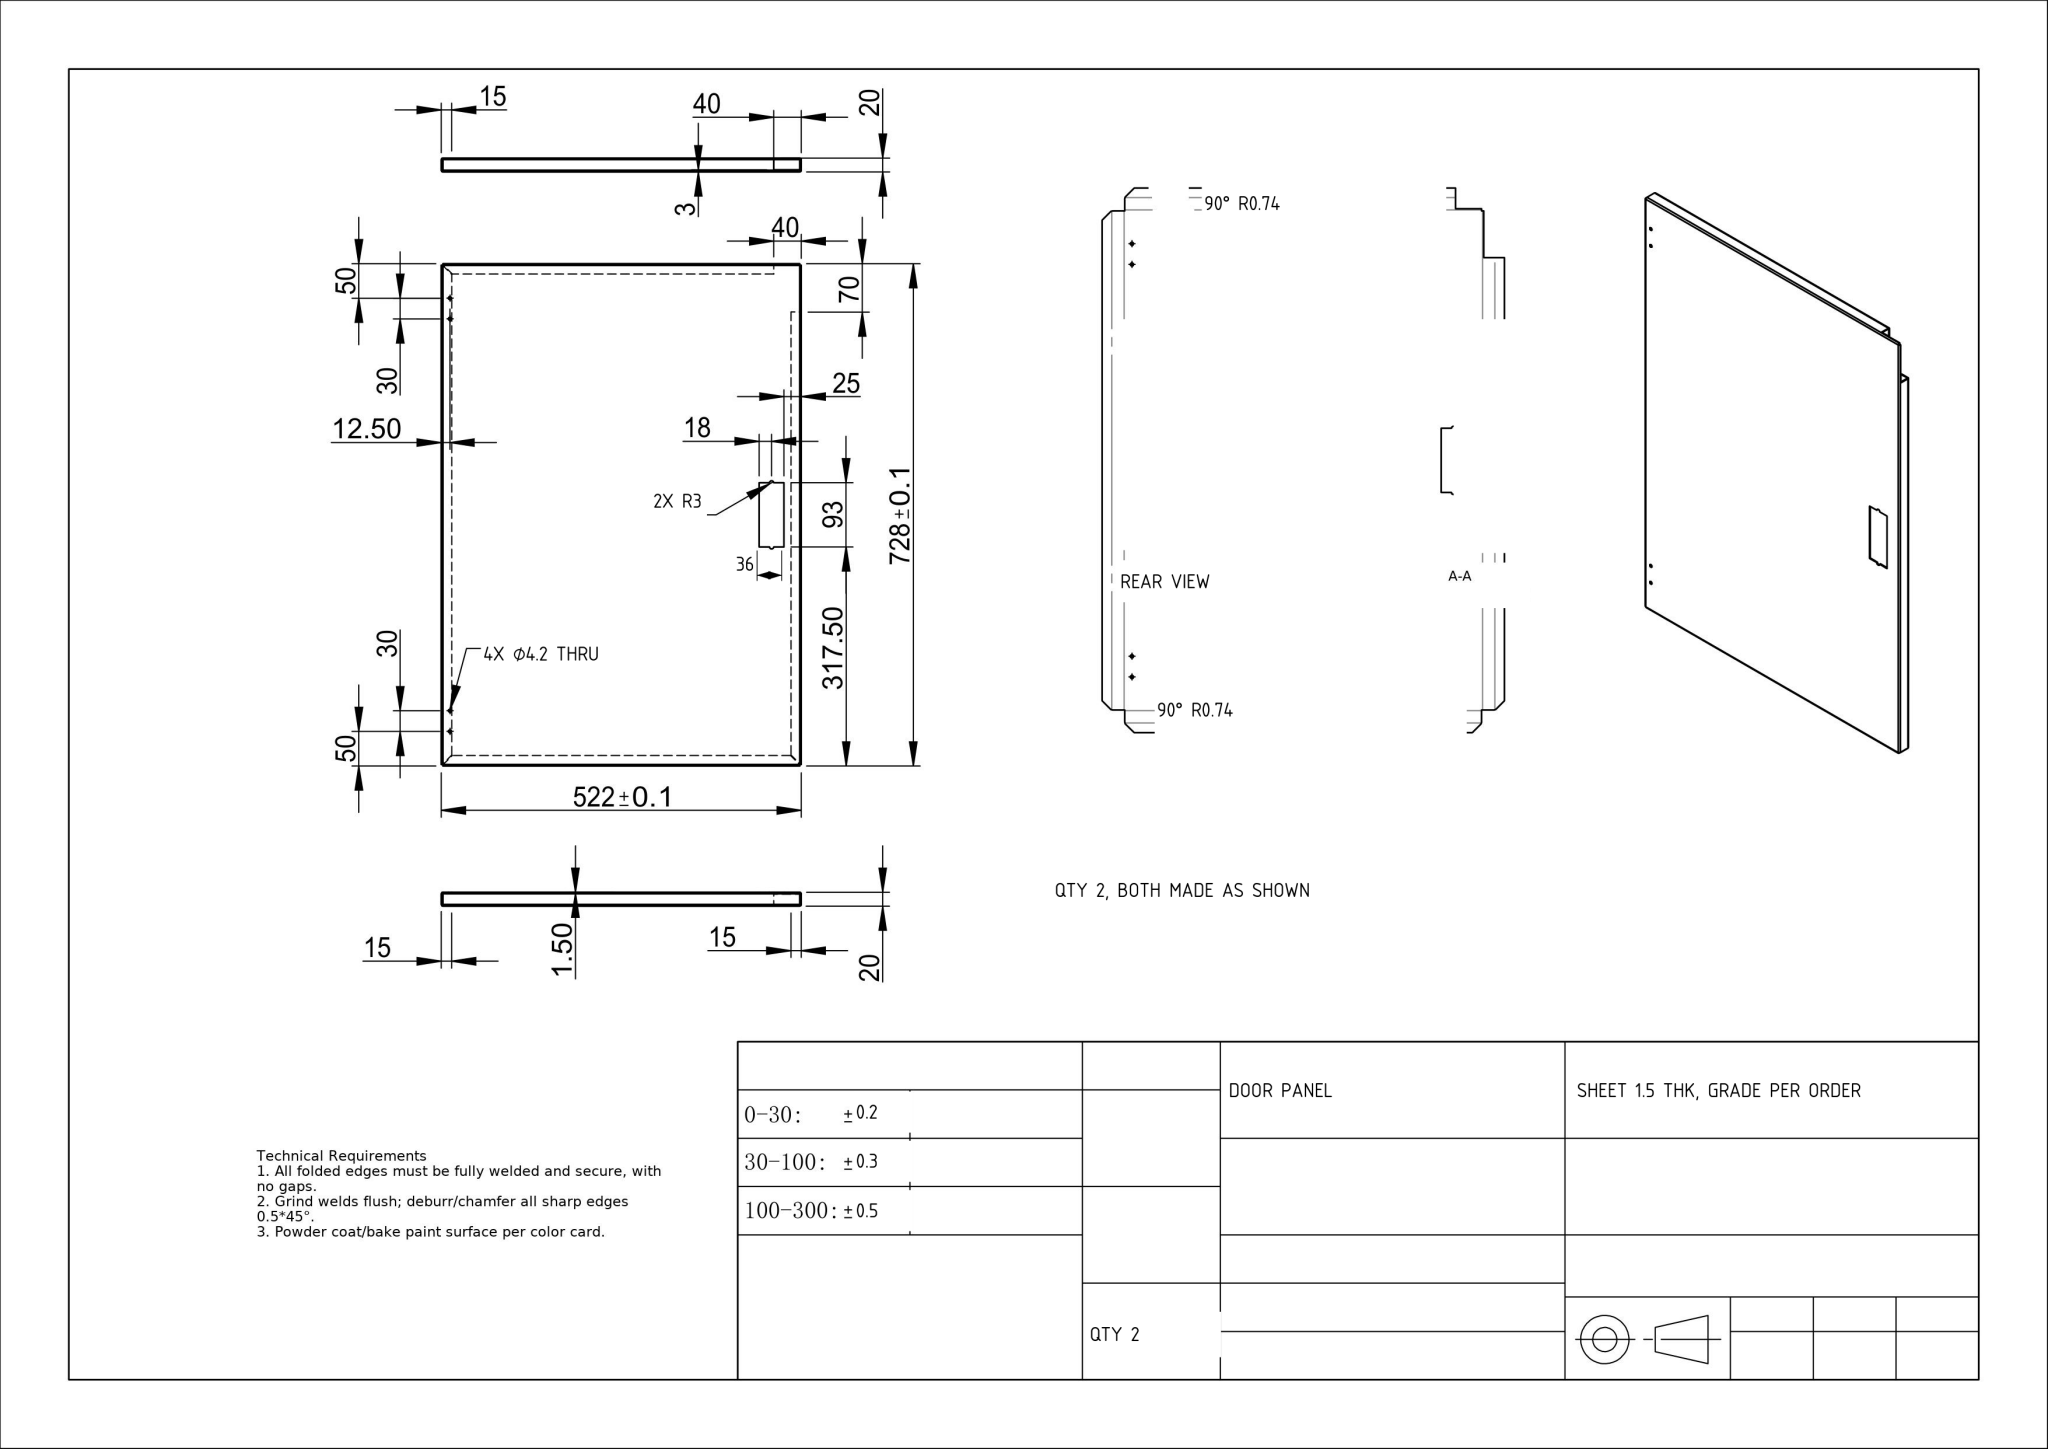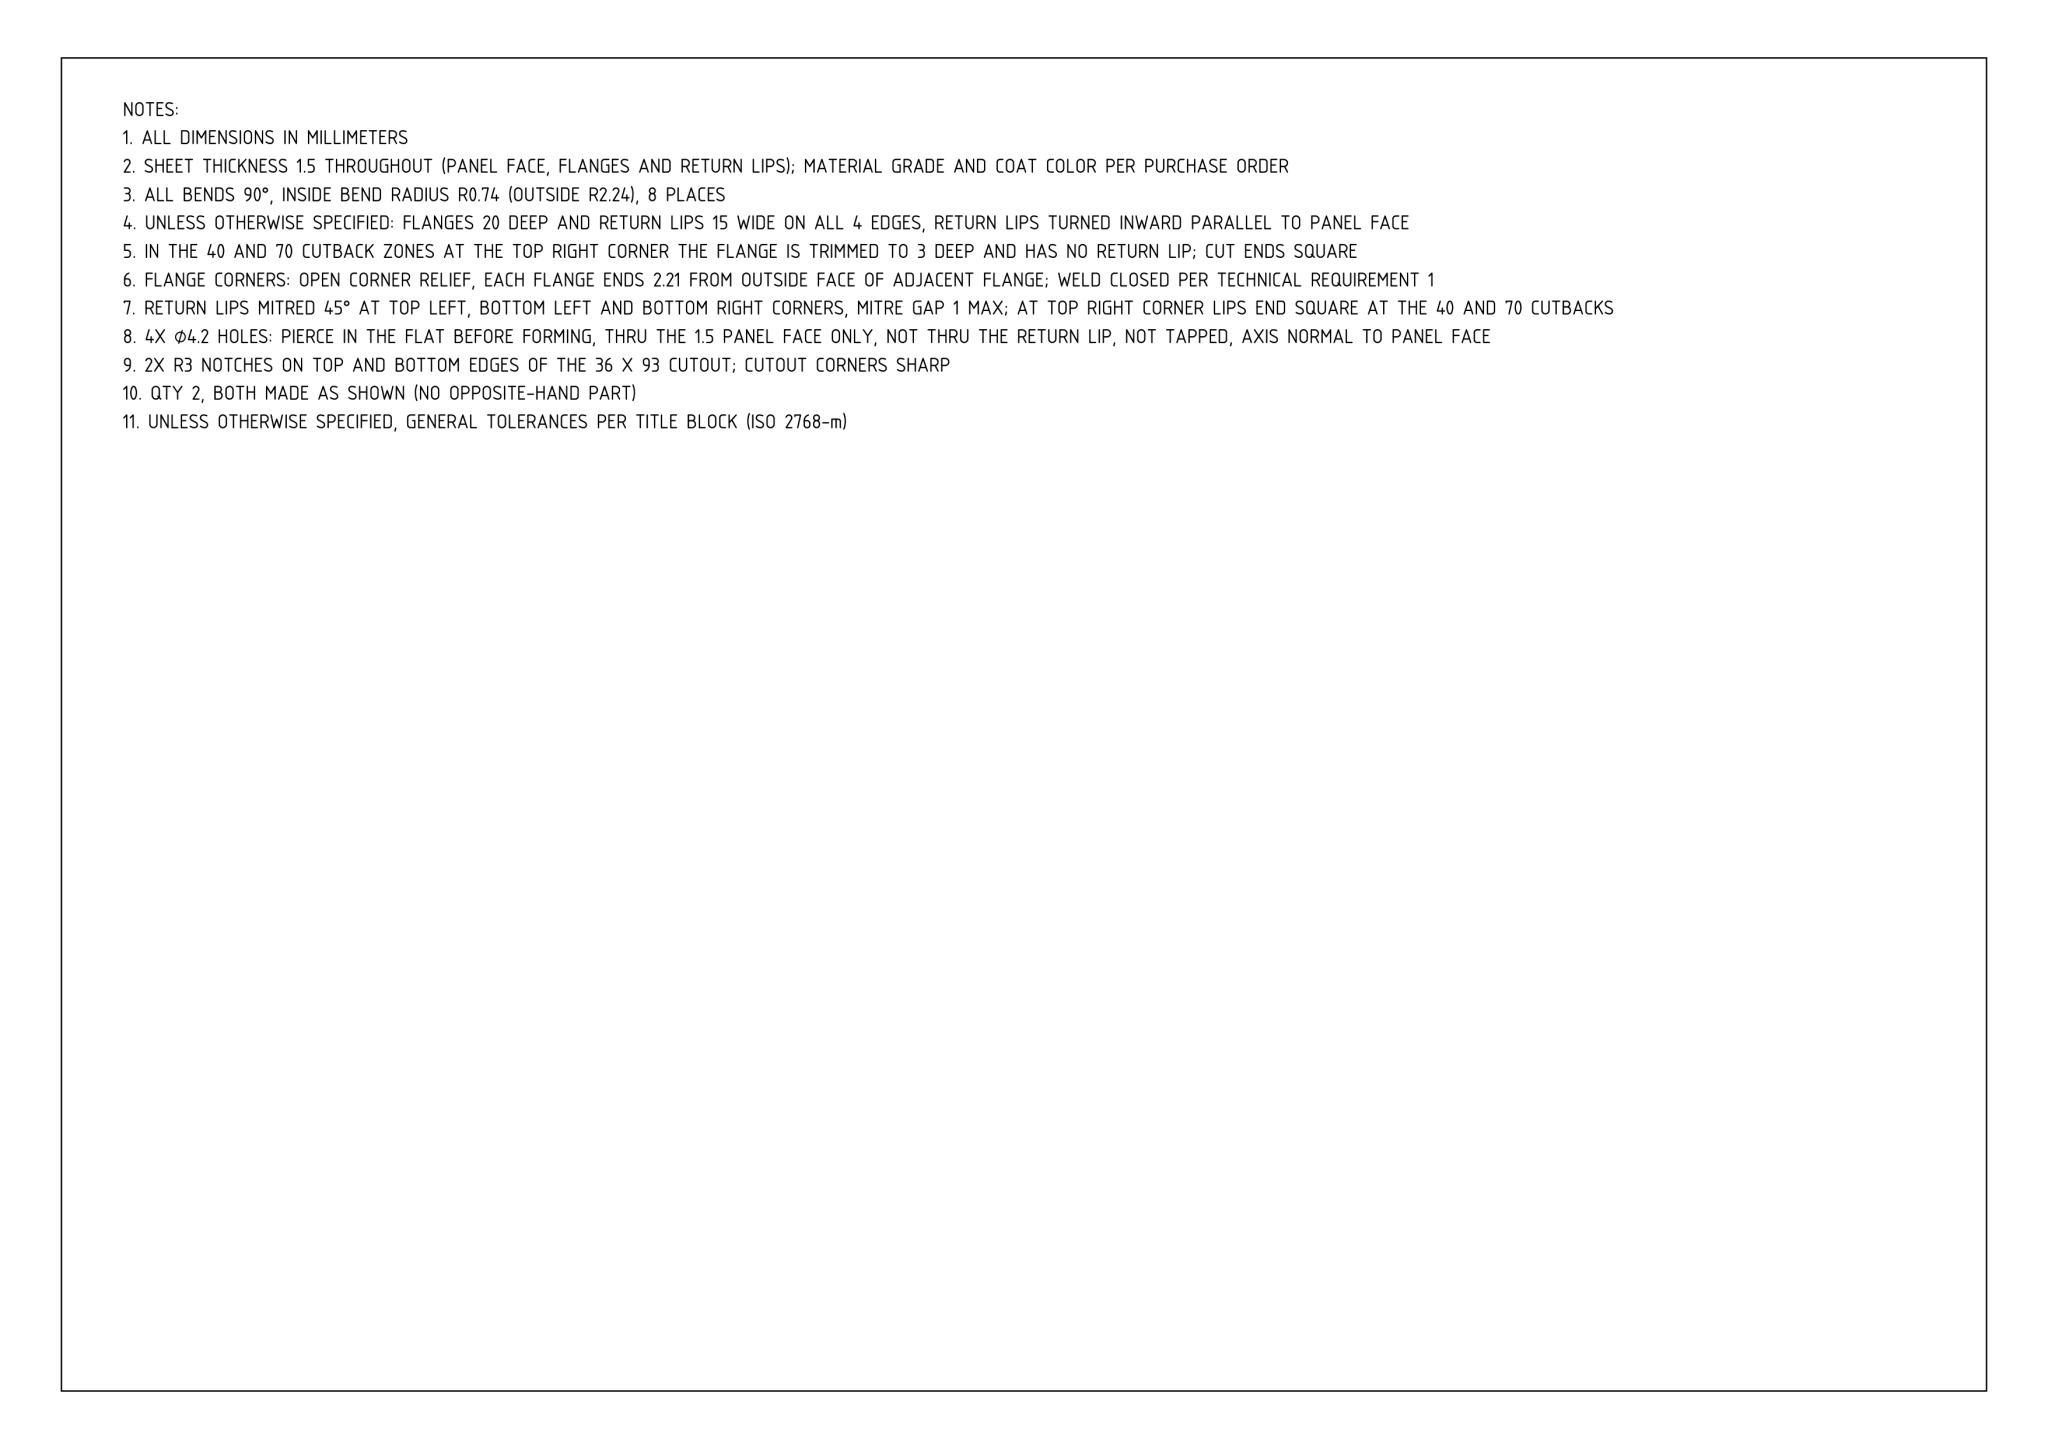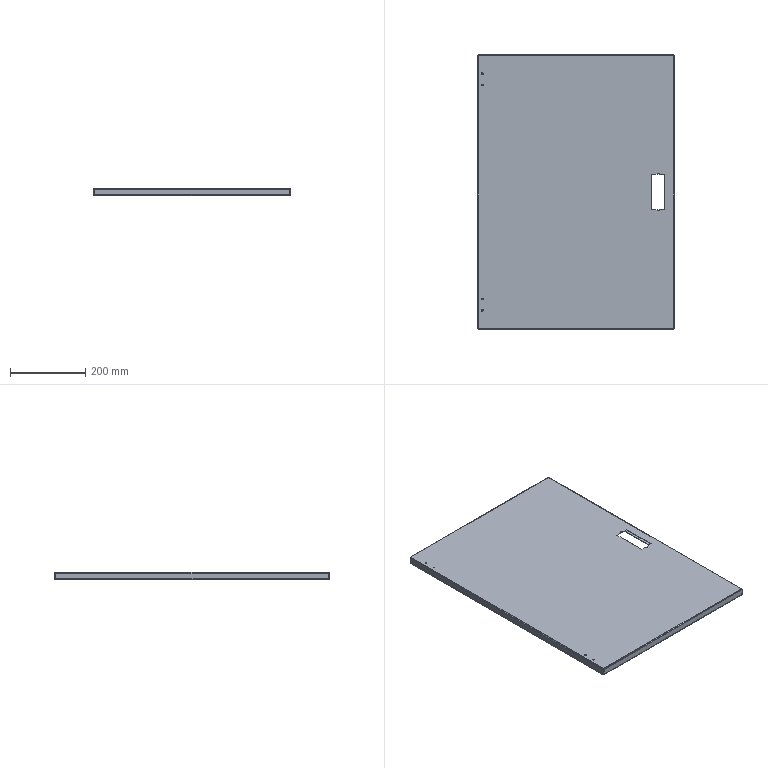Part | NX | mm | 1 solid | 86 faces | box 522 x 728 x 20 mm | volume 673693 mm3 | plane 46 | cylinder 26 | spline 14 | commonest cylinder face diameters 4.2 x8 4.473 x8 1.473 x8 6 x2